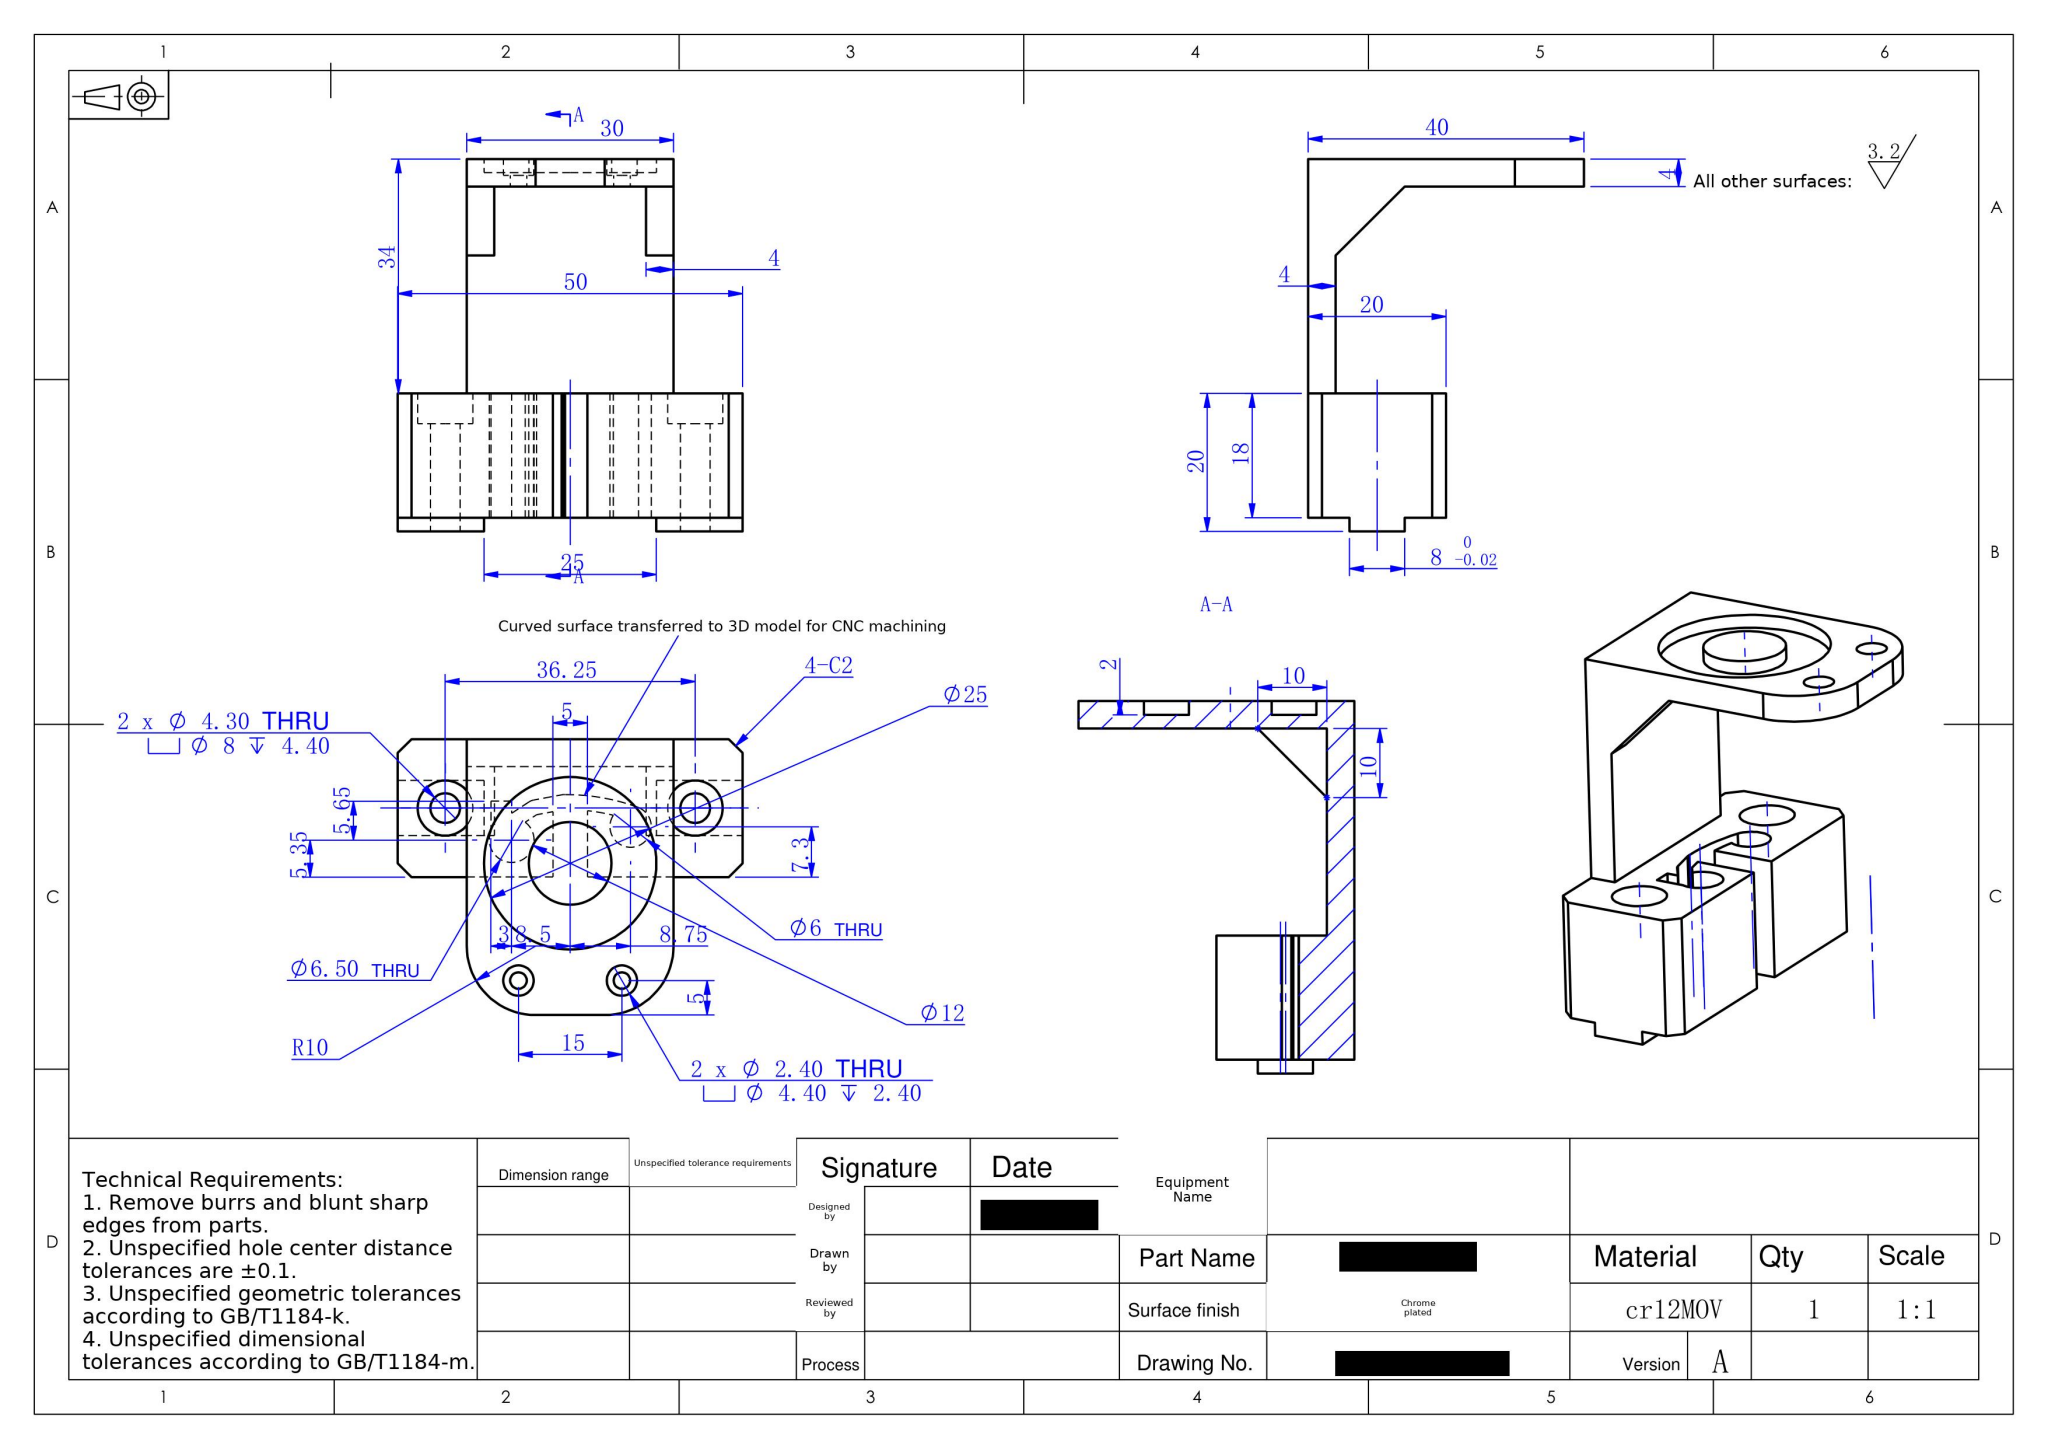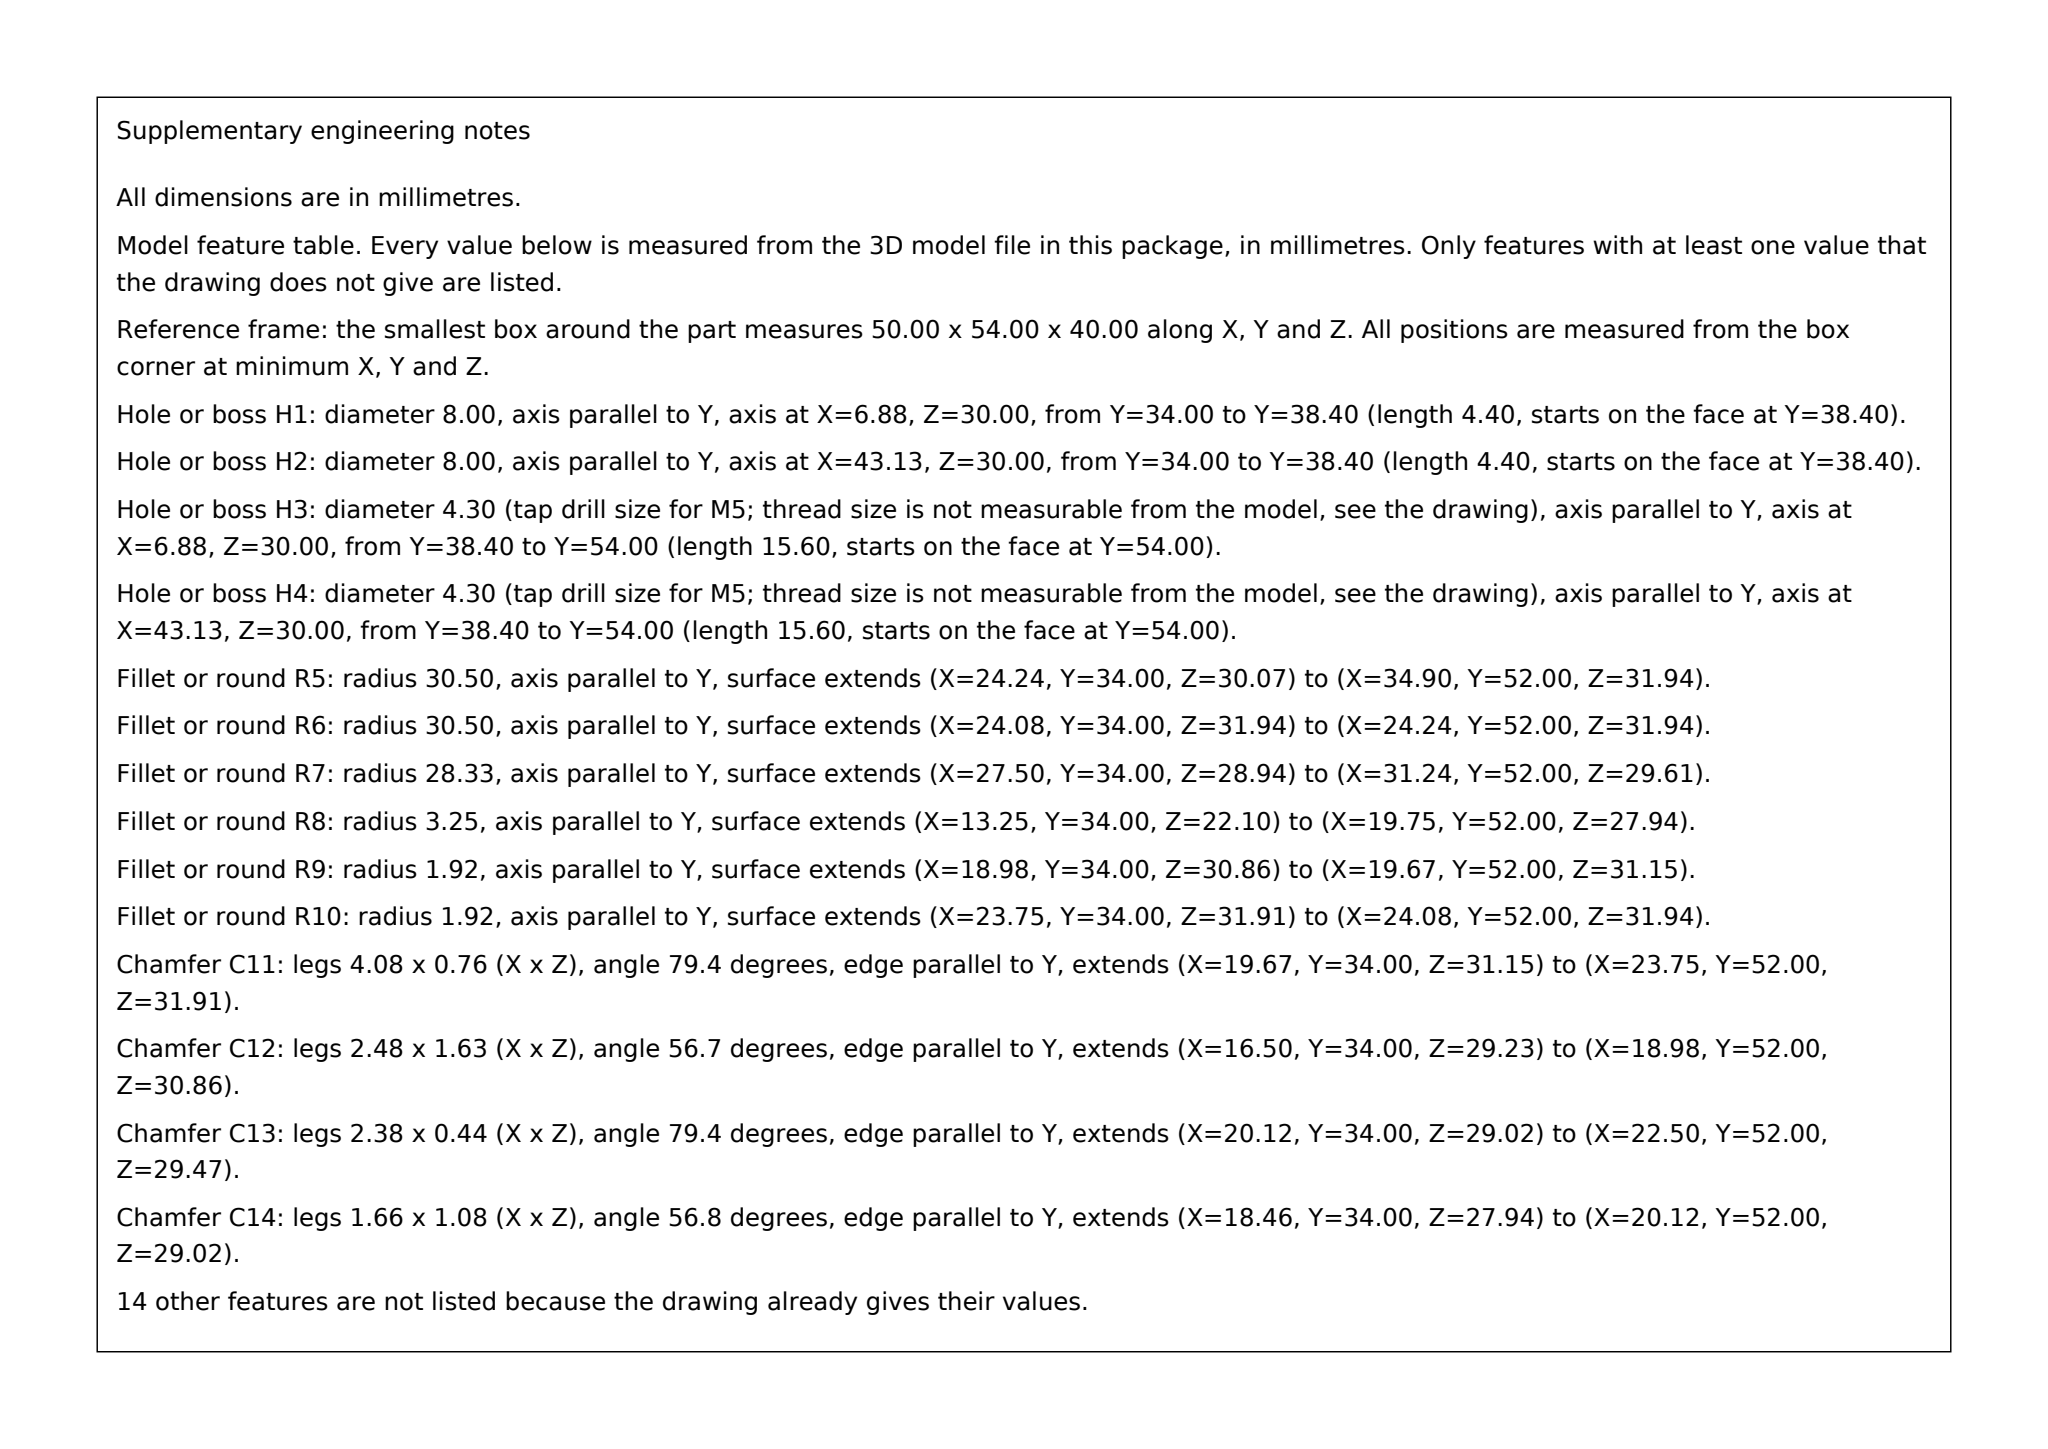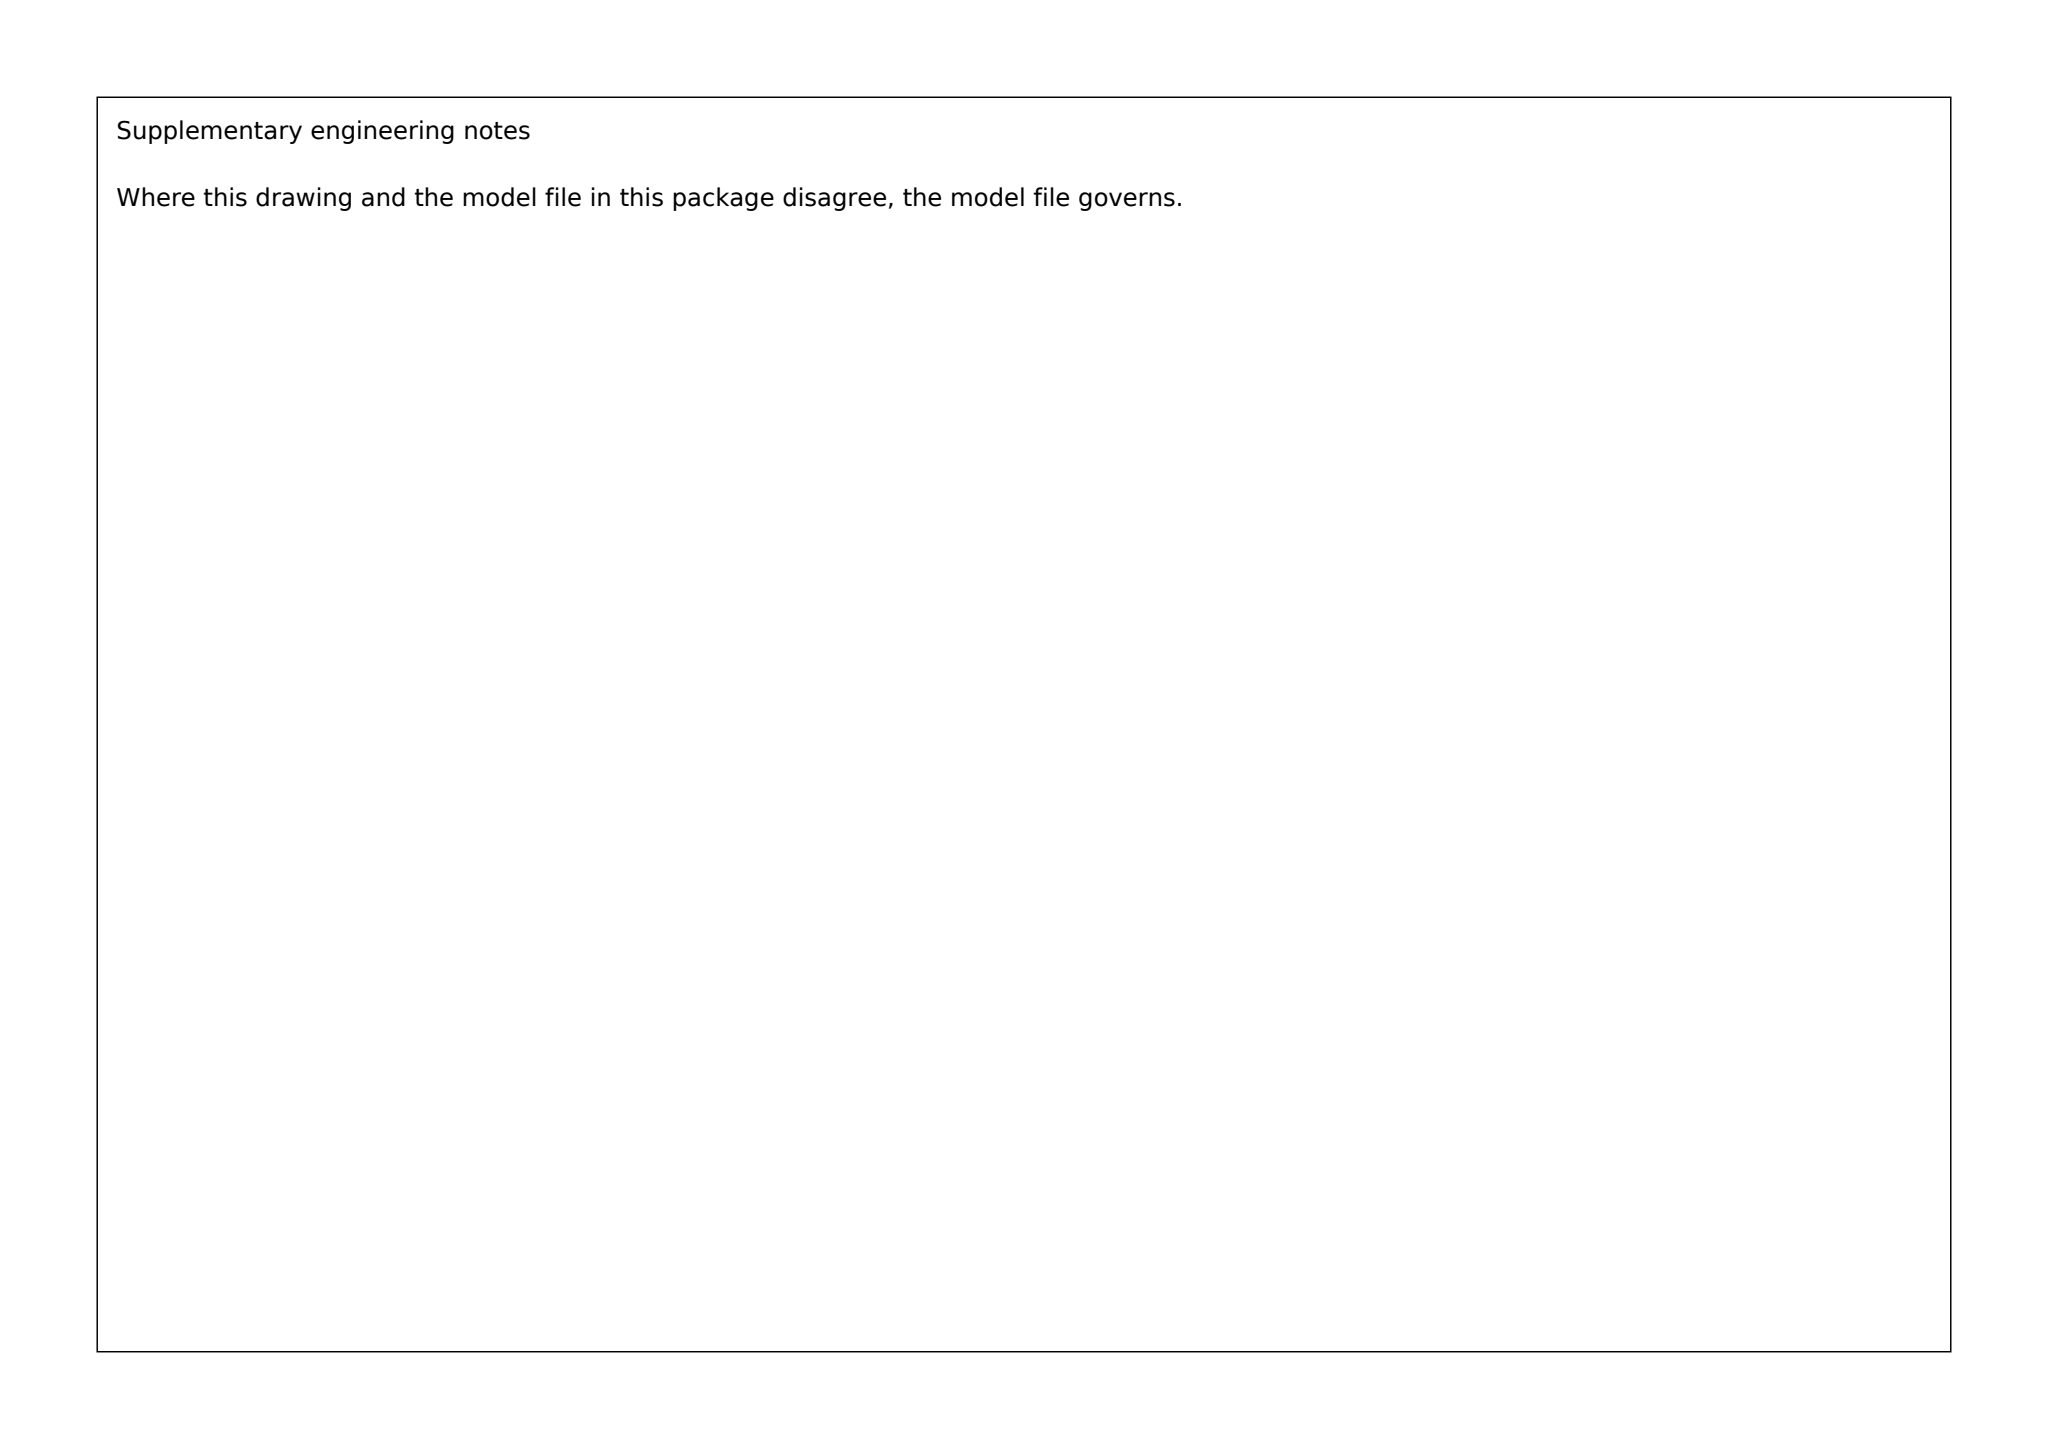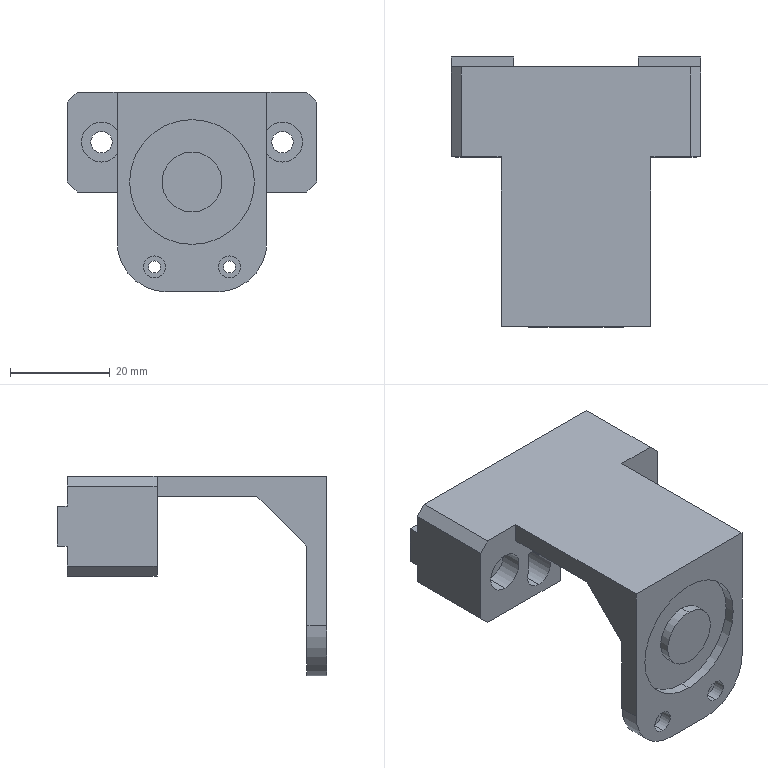Part | SolidWorks | mm | material cr12MOV | 1 solid | 75 faces | box 50 x 54 x 40 mm | volume 22400 mm3 | plane 44 | cylinder 31 | commonest cylinder face diameters 4.4 x4 2.4 x4 8 x4 4.3 x4 12 x2 25 x2 6.5 x2 6 x2
build123d program:
from build123d import *

# Parameters (mm, degrees)
SKETCH1_W                                       = 35
SKETCH1_H                                       = 18
BOSS_EXTRUDE1_DEPTH                             = 20
CUT_EXTRUDE2_DEPTH                              = 88.032
SKETCH3_W                                       = 5
SKETCH3_H                                       = 12.572
CUT_EXTRUDE3_DEPTH                              = 88.032
SKETCH4_W                                       = 3
SKETCH4_H                                       = 5
CUT_EXTRUDE4_DEPTH                              = 88.032
SKETCH5_W                                       = 20
SKETCH5_H                                       = 18
BOSS_EXTRUDE2_DEPTH                             = 7.5
SKETCH6_W                                       = 20
SKETCH6_H                                       = 18
BOSS_EXTRUDE3_DEPTH                             = 7.5
BOSS_EXTRUDE4_REACH                             = 105.604
SKETCH7_W                                       = 13.75
SKETCH7_H                                       = 2
SKETCH8_W                                       = 25
SKETCH8_H                                       = 2
CUT_EXTRUDE5_DEPTH                              = 105.522
SKETCH9_W                                       = 6
SKETCH9_H                                       = 2
CUT_EXTRUDE6_DEPTH                              = 73.64
M4_HEX_SOCKET_HEAD_CAP_SCREW_CBORE1_D           = 4.3
M4_HEX_SOCKET_HEAD_CAP_SCREW_CBORE1_CBORE_D     = 8
M4_HEX_SOCKET_HEAD_CAP_SCREW_CBORE1_CBORE_DEPTH = 4.4
CHAMFER1_SIZE                                   = 2
SKETCH12_W                                      = 30
SKETCH12_H                                      = 30
BOSS_EXTRUDE5_DEPTH                             = 4
SKETCH13_W                                      = 30
SKETCH13_H                                      = 40
BOSS_EXTRUDE6_DEPTH                             = 4
BOSS_EXTRUDE7_DEPTH                             = 4
BOSS_EXTRUDE8_DEPTH                             = 4
FILLET1_R                                       = 10
SKETCH16_R                                      = 12.5
CUT_EXTRUDE7_DEPTH                              = 2
M2_HEX_SOCKET_HEAD_CAP_SCREW_CBORE1_D           = 2.4
M2_HEX_SOCKET_HEAD_CAP_SCREW_CBORE1_CBORE_D     = 4.4
M2_HEX_SOCKET_HEAD_CAP_SCREW_CBORE1_CBORE_DEPTH = 2.4
SKETCH20_R                                      = 6
BOSS_EXTRUDE9_DEPTH                             = 2


with BuildPart() as part:
    # Sketch1 → Boss-Extrude1 (new body)
    with BuildSketch(Plane.XY):
        with Locations((-65.268, 37.75)):
            Rectangle(SKETCH1_W, SKETCH1_H)
    extrude(amount=BOSS_EXTRUDE1_DEPTH)

    # Sketch2 → Cut-Extrude2 (cut, through all)
    with BuildSketch(Plane(origin=(0, 28.75, 0), x_dir=(-1, 0, 0), z_dir=(0, -1, 0))):
        with BuildLine():
            Line((70.597, -11.149), (66.518, -11.909))
            ThreePointArc((66.518, -11.909), (66.354, -11.933), (66.189, -11.942))
            ThreePointArc((66.189, -11.942), (66.109, -11.942), (66.029, -11.943))
            ThreePointArc((66.029, -11.943), (60.614, -11.484), (55.367, -10.071))
            ThreePointArc((55.367, -10.071), (55.636, -4.433), (59.027, -8.944))
            ThreePointArc((59.027, -8.944), (62.495, -9.576), (66.015, -9.773))
            ThreePointArc((66.015, -9.773), (66.078, -9.773), (66.142, -9.772))
            Line((66.142, -9.772), (70.15, -9.025))
            Line((70.15, -9.025), (71.805, -7.944))
            ThreePointArc((71.805, -7.944), (73.759, -2.104), (75.746, -7.933))
            Line((75.746, -7.933), (71.289, -10.861))
            ThreePointArc((71.289, -10.861), (70.957, -11.039), (70.597, -11.149))
        make_face()
    extrude(amount=-CUT_EXTRUDE2_DEPTH, mode=Mode.SUBTRACT)

    # Sketch3 → Cut-Extrude3 (cut, through all)
    with BuildSketch(Plane(origin=(0, 46.75, 0), x_dir=(1, 0, 0), z_dir=(0, 1, 0))):
        with Locations((-65.268, -4.073)):
            Rectangle(SKETCH3_W, SKETCH3_H)
    extrude(amount=-CUT_EXTRUDE3_DEPTH, mode=Mode.SUBTRACT)

    # Sketch4 → Cut-Extrude4 (cut, through all)
    with BuildSketch(Plane(origin=(0, 28.75, 0), x_dir=(-1, 0, 0), z_dir=(0, -1, 0))):
        with Locations((75.268, -8.5)):
            Rectangle(SKETCH4_W, SKETCH4_H)
    extrude(amount=-CUT_EXTRUDE4_DEPTH, mode=Mode.SUBTRACT)

    # Sketch5 → Boss-Extrude2 (add)
    with BuildSketch(Plane(origin=(-47.768, 0, 0), x_dir=(0, 0, -1), z_dir=(1, 0, 0))):
        with Locations((-10, 37.75)):
            Rectangle(SKETCH5_W, SKETCH5_H)
    extrude(amount=BOSS_EXTRUDE2_DEPTH)

    # Sketch6 → Boss-Extrude3 (add)
    with BuildSketch(Plane.ZY.offset(82.768)):
        with Locations((10, 37.75)):
            Rectangle(SKETCH6_W, SKETCH6_H)
    extrude(amount=BOSS_EXTRUDE3_DEPTH)

    # Boss-Extrude4: up to this face of the body (flat: up to its plane)
    boss_extrude4_end = Plane(part.part.faces().sort_by_distance((-65.268, 37.75, 20))[0])
    # Sketch7 → Boss-Extrude4 (add, up to the picked face)
    with BuildSketch(Plane(origin=(0, 0, 0), x_dir=(-1, 0, 0), z_dir=(0, 0, -1)), mode=Mode.PRIVATE) as boss_extrude4_sk1:
        with Locations((83.393, 47.75)):
            Rectangle(SKETCH7_W, SKETCH7_H)
    boss_extrude4_tool1 = split(extrude(boss_extrude4_sk1.sketch, amount=-BOSS_EXTRUDE4_REACH, mode=Mode.PRIVATE), bisect_by=boss_extrude4_end, keep=Keep.BOTH, mode=Mode.PRIVATE)
    # Sketch7 → Boss-Extrude4 (add, up to the picked face)
    with BuildSketch(Plane(origin=(0, 0, 0), x_dir=(-1, 0, 0), z_dir=(0, 0, -1)), mode=Mode.PRIVATE) as boss_extrude4_sk2:
        with Locations((47.143, 47.75)):
            Rectangle(SKETCH7_W, SKETCH7_H)
    boss_extrude4_tool2 = split(extrude(boss_extrude4_sk2.sketch, amount=-BOSS_EXTRUDE4_REACH, mode=Mode.PRIVATE), bisect_by=boss_extrude4_end, keep=Keep.BOTH, mode=Mode.PRIVATE)
    add(boss_extrude4_tool1.solids().sort_by(Axis((-83.393, 47.75, 0), (0, 0, 1)))[0])
    add(boss_extrude4_tool2.solids().sort_by(Axis((-47.143, 47.75, 0), (0, 0, 1)))[0])

    # Sketch8 → Cut-Extrude5 (cut, through all)
    with BuildSketch(Plane(origin=(0, 0, 0), x_dir=(-1, 0, 0), z_dir=(0, 0, -1))):
        with Locations((65.268, 47.75)):
            Rectangle(SKETCH8_W, SKETCH8_H)
    extrude(amount=-CUT_EXTRUDE5_DEPTH, mode=Mode.SUBTRACT)

    # Sketch9 → Cut-Extrude6 (cut, through all)
    with BuildSketch(Plane(origin=(-40.268, 0, 0), x_dir=(0, 0, -1), z_dir=(1, 0, 0))):
        with Locations((-17, 47.75)):
            Rectangle(SKETCH9_W, SKETCH9_H)
        with Locations((-3, 47.75)):
            Rectangle(SKETCH9_W, SKETCH9_H)
    extrude(amount=-CUT_EXTRUDE6_DEPTH, mode=Mode.SUBTRACT)

    # M4 Hex Socket Head Cap Screw CBORE1 (through all)
    with Locations(Plane(origin=(0, 28.75, 0), x_dir=(-1, 0, 0), z_dir=(0, -1, 0))):
        with Locations((83.393, -10), (47.143, -10)):
            CounterBoreHole(M4_HEX_SOCKET_HEAD_CAP_SCREW_CBORE1_D / 2, M4_HEX_SOCKET_HEAD_CAP_SCREW_CBORE1_CBORE_D / 2, M4_HEX_SOCKET_HEAD_CAP_SCREW_CBORE1_CBORE_DEPTH)

    # Chamfer1
    chamfer1_edges = [part.edges().sort_by_distance(p)[0] for p in [
        (-90.268, 37.75, 0),
        (-40.268, 37.75, 0),
        (-90.268, 37.75, 20),
        (-40.268, 37.75, 20),
    ]]
    chamfer(chamfer1_edges, length=CHAMFER1_SIZE)

    # Sketch12 → Boss-Extrude5 (add)
    with BuildSketch(Plane.XY.offset(20)):
        with Locations((-65.268, 13.75)):
            Rectangle(SKETCH12_W, SKETCH12_H)
    extrude(amount=-BOSS_EXTRUDE5_DEPTH)

    # Sketch13 → Boss-Extrude6 (add)
    with BuildSketch(Plane.XZ.offset(1.25)):
        with Locations((-65.268, 0)):
            Rectangle(SKETCH13_W, SKETCH13_H)
    extrude(amount=BOSS_EXTRUDE6_DEPTH)

    # Sketch14 → Boss-Extrude7 (add)
    with BuildSketch(Plane.ZY.offset(80.268)):
        Polygon((16, 8.75), (6, -1.25), (16, -1.25), align=None)
    extrude(amount=-BOSS_EXTRUDE7_DEPTH)

    # Sketch15 → Boss-Extrude8 (add)
    with BuildSketch(Plane(origin=(-50.268, 0, 0), x_dir=(0, 0, -1), z_dir=(1, 0, 0))):
        Polygon((-16, -1.25), (-16, 8.75), (-6, -1.25), align=None)
    extrude(amount=-BOSS_EXTRUDE8_DEPTH)

    # Fillet1
    fillet1_edges = [part.edges().sort_by_distance(p)[0] for p in [
        (-80.268, -3.25, -20),
        (-50.268, -3.25, -20),
    ]]
    fillet(fillet1_edges, radius=FILLET1_R)

    # Sketch16 → Cut-Extrude7 (cut)
    with BuildSketch(Plane.XZ.offset(5.25)):
        with Locations(Location((-65.268, 2, 0), (0, 0, 270))):
            Circle(SKETCH16_R)
    extrude(amount=-CUT_EXTRUDE7_DEPTH, mode=Mode.SUBTRACT)

    # M2 Hex Socket Head Cap Screw CBORE1 (through all)
    with Locations(Plane(origin=(0, -5.25, 0), x_dir=(-1, 0, 0), z_dir=(0, -1, 0))):
        with Locations((57.768, 15), (72.768, 15)):
            CounterBoreHole(M2_HEX_SOCKET_HEAD_CAP_SCREW_CBORE1_D / 2, M2_HEX_SOCKET_HEAD_CAP_SCREW_CBORE1_CBORE_D / 2, M2_HEX_SOCKET_HEAD_CAP_SCREW_CBORE1_CBORE_DEPTH)

    # Sketch20 → Boss-Extrude9 (add)
    with BuildSketch(Plane.XZ.offset(3.25)):
        with Locations(Location((-65.268, 2, 0), (0, 0, 270))):
            Circle(SKETCH20_R)
    extrude(amount=BOSS_EXTRUDE9_DEPTH)


solid = part.part